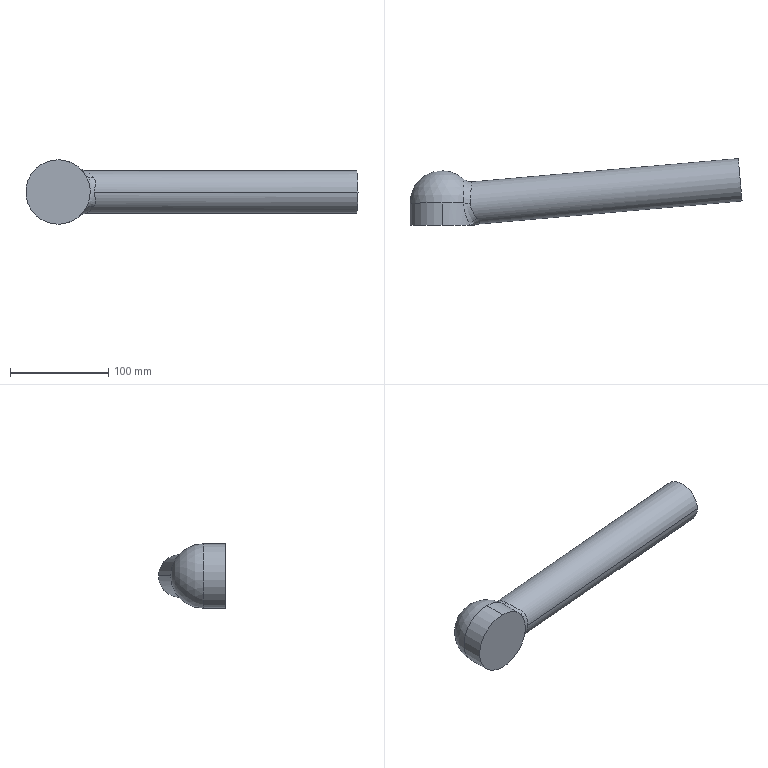Component | SolidWorks | RehabilitationChair-18-6-2 | 1 solid | 12 faces | volume 559517 mm3 | cylinder 5 | spline 4 | plane 2 | sphere 1 | commonest cylinder face diameters 65.746 x3 43.427 x2